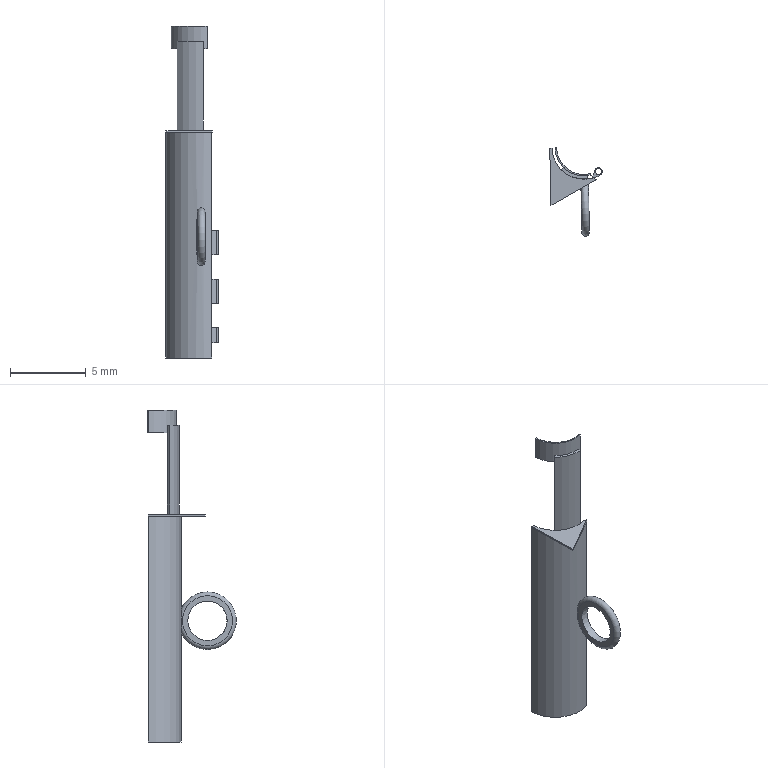Component | NX | FINGER_HOLDER | 4 solids | 50 faces | volume 15 mm3 | plane 28 | cylinder 21 | torus 1 | commonest cylinder face diameters 4.2 x3 3.8 x3 1.1 x3 4.197 x3 0.5 x3 0.4 x3 4.5 x1 2.6 x1